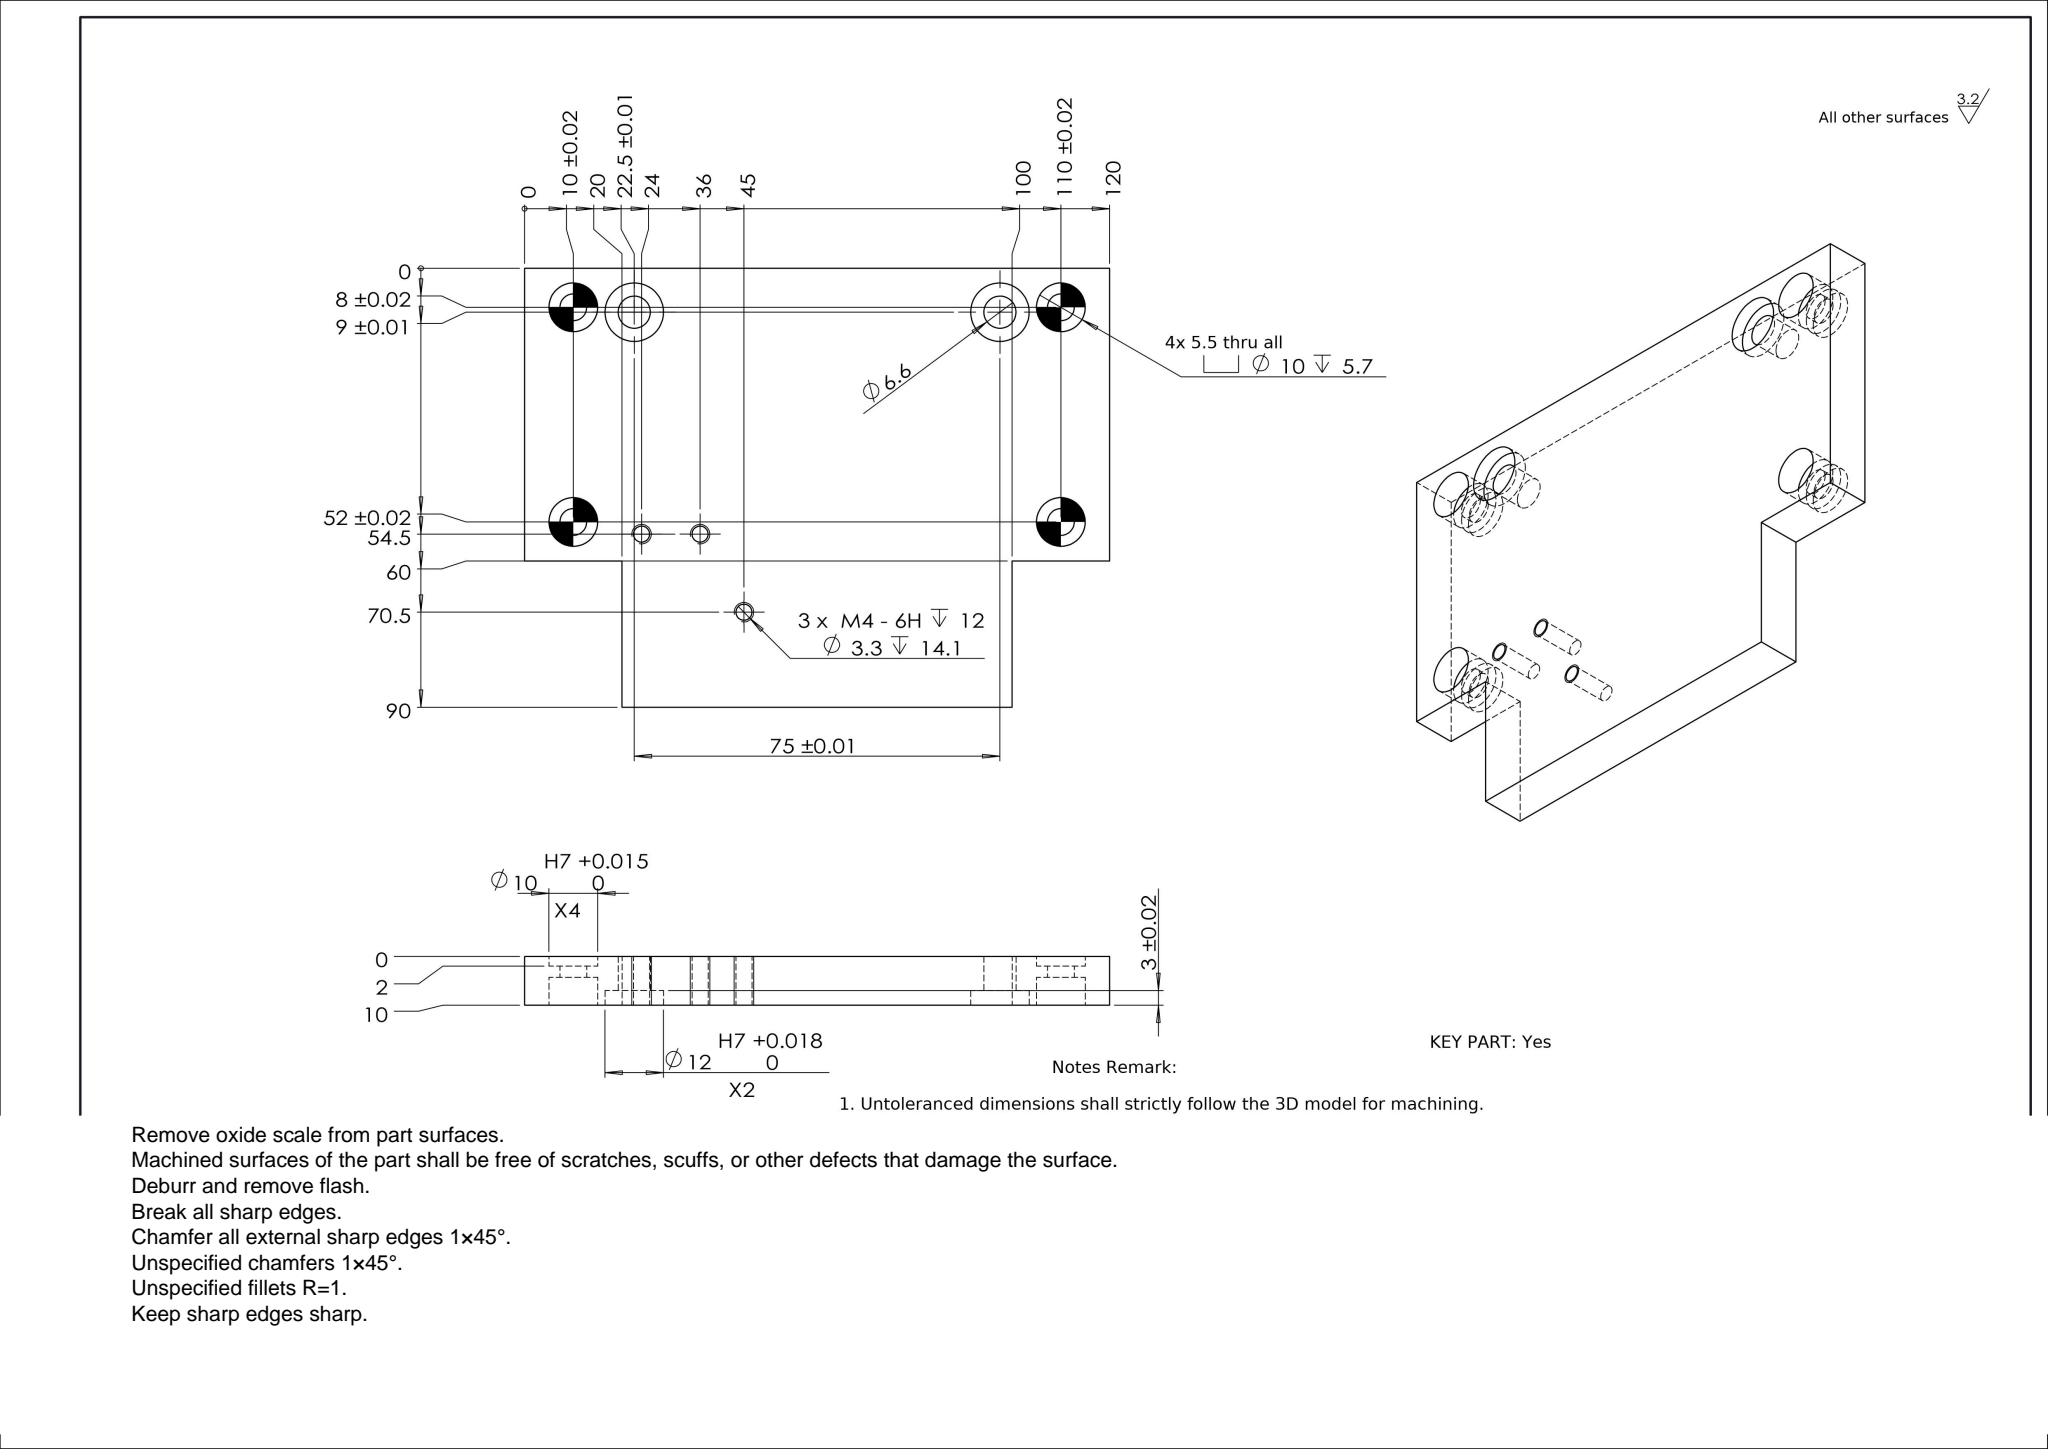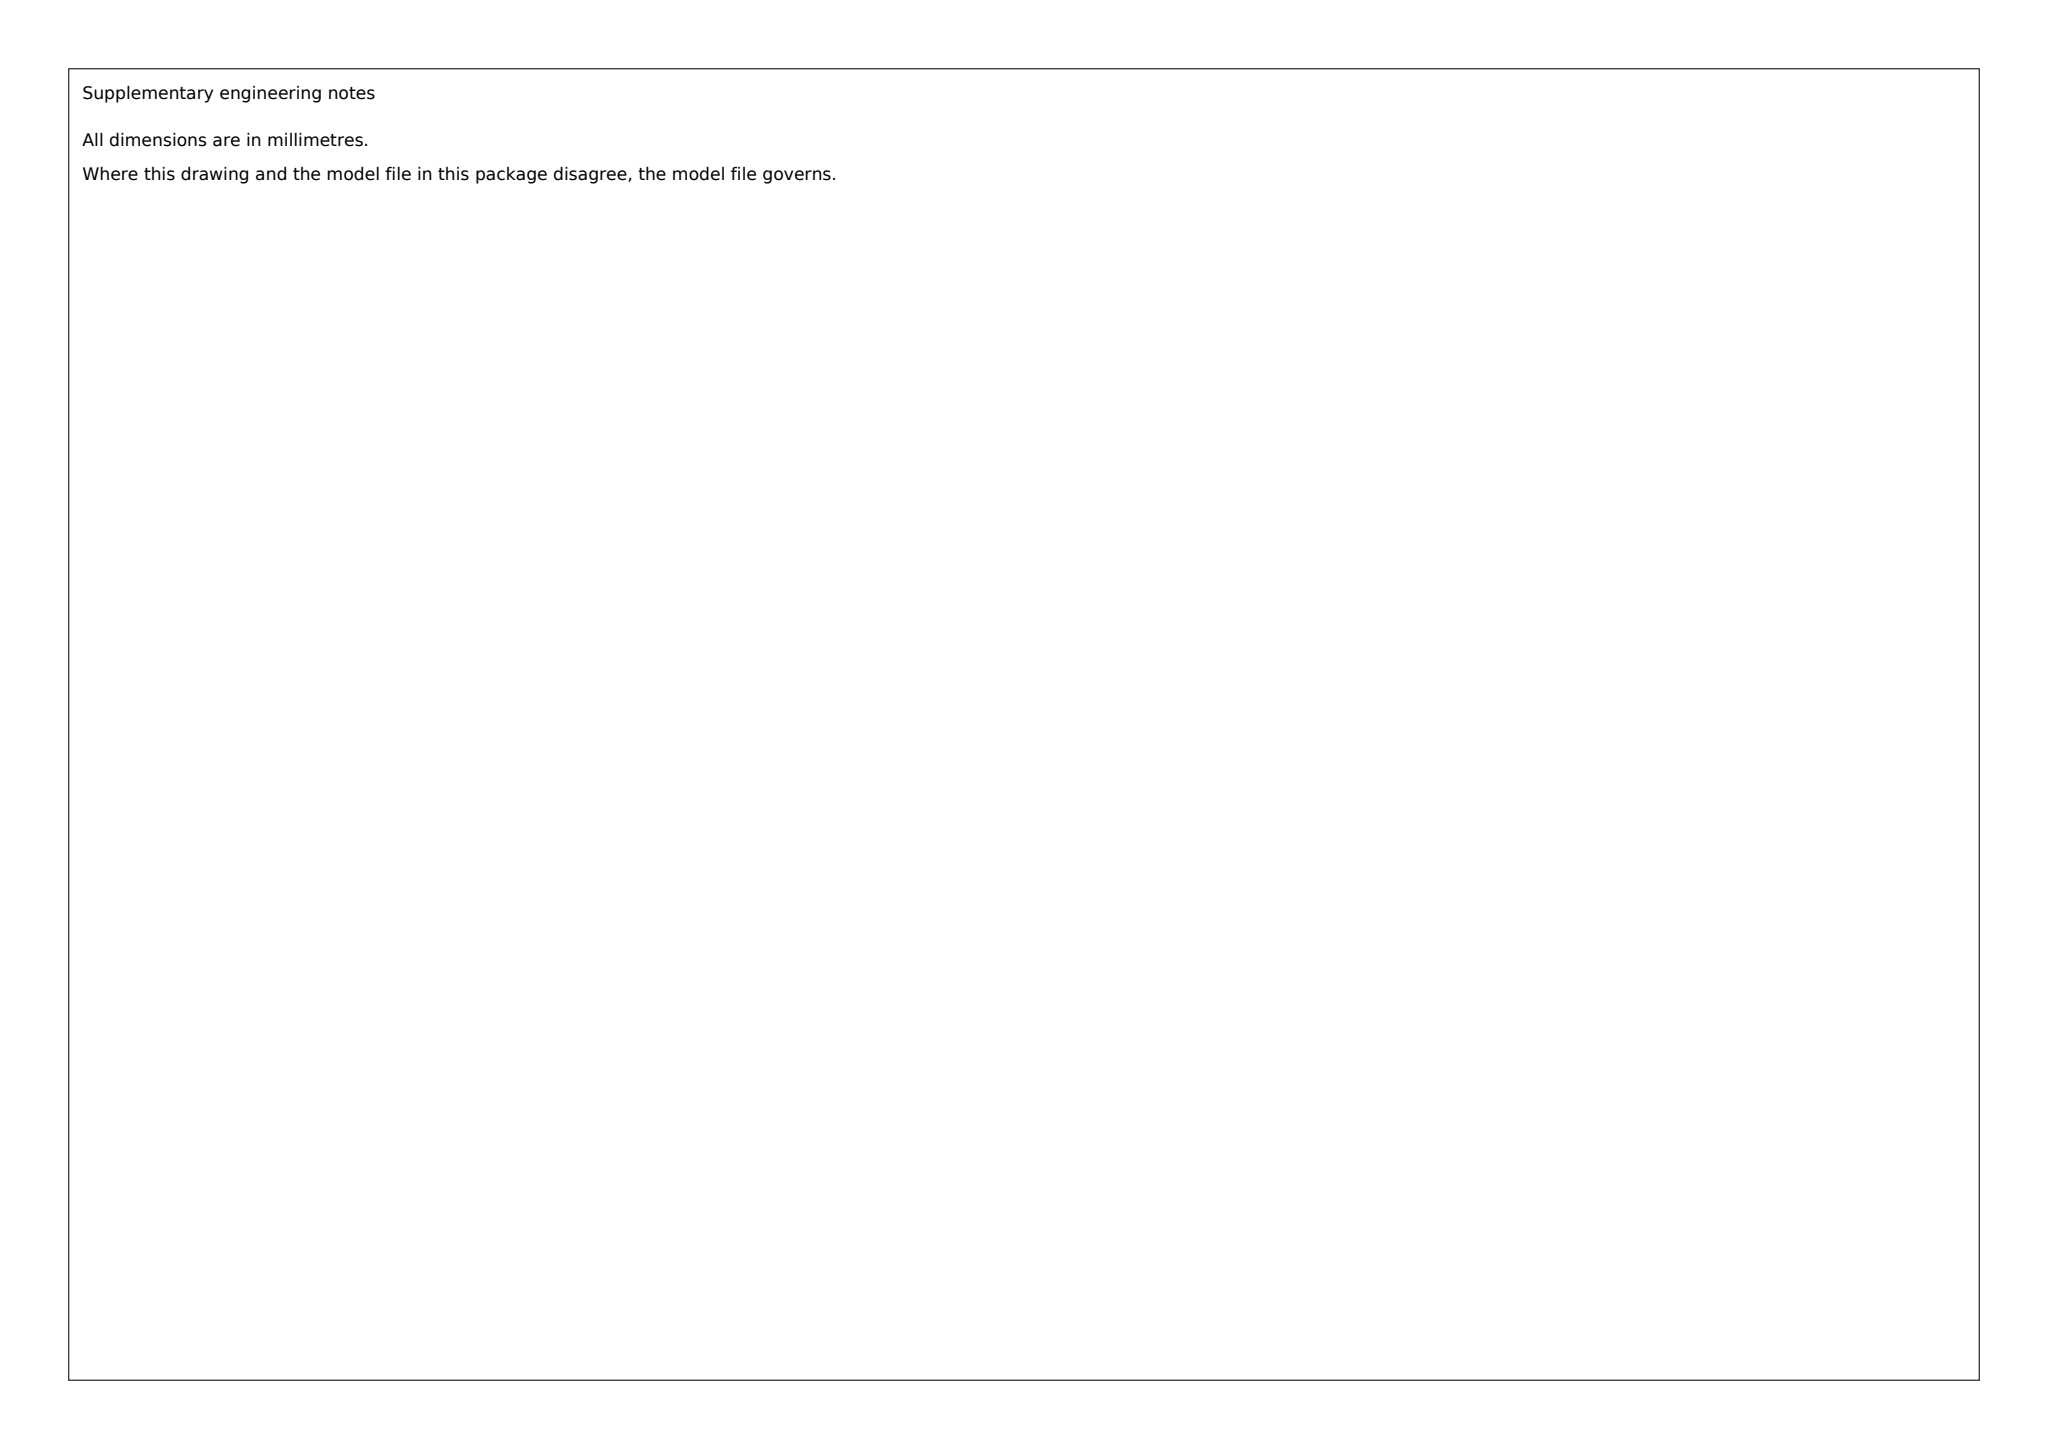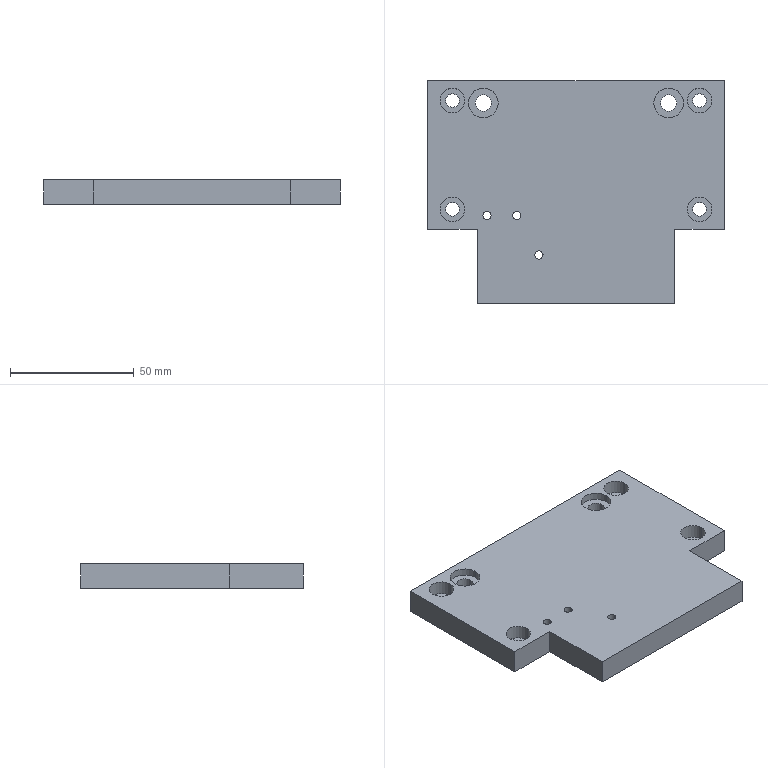Part | SolidWorks | mm | 1 solid | 58 faces | box 120 x 90 x 10 mm | volume 91948 mm3 | cylinder 38 | plane 20 | commonest cylinder face diameters 10 x16 5.5 x8 3.3 x6 6.6 x4 12 x4
build123d program:
from build123d import *

# Parameters (mm, degrees)
SKETCH1_W                                         = 120
SKETCH1_H                                         = 60
BOSS_EXTRUDE1_DEPTH                               = 10
SKETCH2_R                                         = 6
CUT_EXTRUDE1_DEPTH                                = 3
HOLE_SIZE_ACCORDING_TO_HEXAGON_SOCKET_D           = 5.5
HOLE_SIZE_ACCORDING_TO_HEXAGON_SOCKET_CBORE_D     = 10
HOLE_SIZE_ACCORDING_TO_HEXAGON_SOCKET_CBORE_DEPTH = 5.7
SKETCH6_W                                         = 80
SKETCH6_H                                         = 30
BOSS_EXTRUDE2_DEPTH                               = 10
SIZE_MM_DOWEL_PIN_HOLE_1_D                        = 10
SIZE_MM_DOWEL_PIN_HOLE_1_DEPTH                    = 2
HOLE_SIZE_ACCORDING_TO_HEXAGON_SO_2_D             = 6.6
M4_TAPPED_HOLE1_D                                 = 3.3
M4_TAPPED_HOLE1_DEPTH                             = 14.1
M4_TAPPED_HOLE1_TIP                               = 0.9914


with BuildPart() as part:
    # Sketch1 → Boss-Extrude1 (new body)
    with BuildSketch(Plane.XY):
        Rectangle(SKETCH1_W, SKETCH1_H)
    extrude(amount=BOSS_EXTRUDE1_DEPTH)

    # Sketch2 → Cut-Extrude1 (cut)
    with BuildSketch(Plane.XY.offset(10)):
        with Locations((-37.5, 21)):
            Circle(SKETCH2_R)
        with Locations((37.5, 21)):
            Circle(SKETCH2_R)
    extrude(amount=-CUT_EXTRUDE1_DEPTH, mode=Mode.SUBTRACT)

    # Hole Size _ according to_ Hexagon Socket (through all)
    with Locations(Plane.XY.offset(10)):
        with Locations((50, 22), (50, -22), (-50, -22), (-50, 22)):
            CounterBoreHole(HOLE_SIZE_ACCORDING_TO_HEXAGON_SOCKET_D / 2, HOLE_SIZE_ACCORDING_TO_HEXAGON_SOCKET_CBORE_D / 2, HOLE_SIZE_ACCORDING_TO_HEXAGON_SOCKET_CBORE_DEPTH)

    # Sketch6 → Boss-Extrude2 (add)
    with BuildSketch(Plane.XY.offset(10)):
        with Locations((0, -45)):
            Rectangle(SKETCH6_W, SKETCH6_H)
    extrude(amount=-BOSS_EXTRUDE2_DEPTH)

    # Size mm Dowel Pin Hole 1
    with Locations(Plane(origin=(0, 0, 0), x_dir=(-1, 0, 0), z_dir=(0, 0, -1))):
        with Locations((-50, 22), (-50, -22), (50, 22), (50, -22)):
            Hole(SIZE_MM_DOWEL_PIN_HOLE_1_D / 2, depth=SIZE_MM_DOWEL_PIN_HOLE_1_DEPTH)

    # Hole Size _ according to_ Hexagon So 2 (through all)
    with Locations(Plane(origin=(0, 0, 0), x_dir=(-1, 0, 0), z_dir=(0, 0, -1))):
        with Locations((37.5, 21), (-37.5, 21)):
            Hole(HOLE_SIZE_ACCORDING_TO_HEXAGON_SO_2_D / 2)

    # M4 Tapped Hole1
    with Locations(Plane.XY.offset(10)):
        with Locations((-36, -24.5), (-24, -24.5), (-15, -40.5)):
            Hole(M4_TAPPED_HOLE1_D / 2, depth=M4_TAPPED_HOLE1_DEPTH)
            with Locations((0, 0, -(M4_TAPPED_HOLE1_DEPTH + M4_TAPPED_HOLE1_TIP / 2))):  # 118° drill point
                Cone(0, M4_TAPPED_HOLE1_D / 2, M4_TAPPED_HOLE1_TIP, mode=Mode.SUBTRACT)


solid = part.part